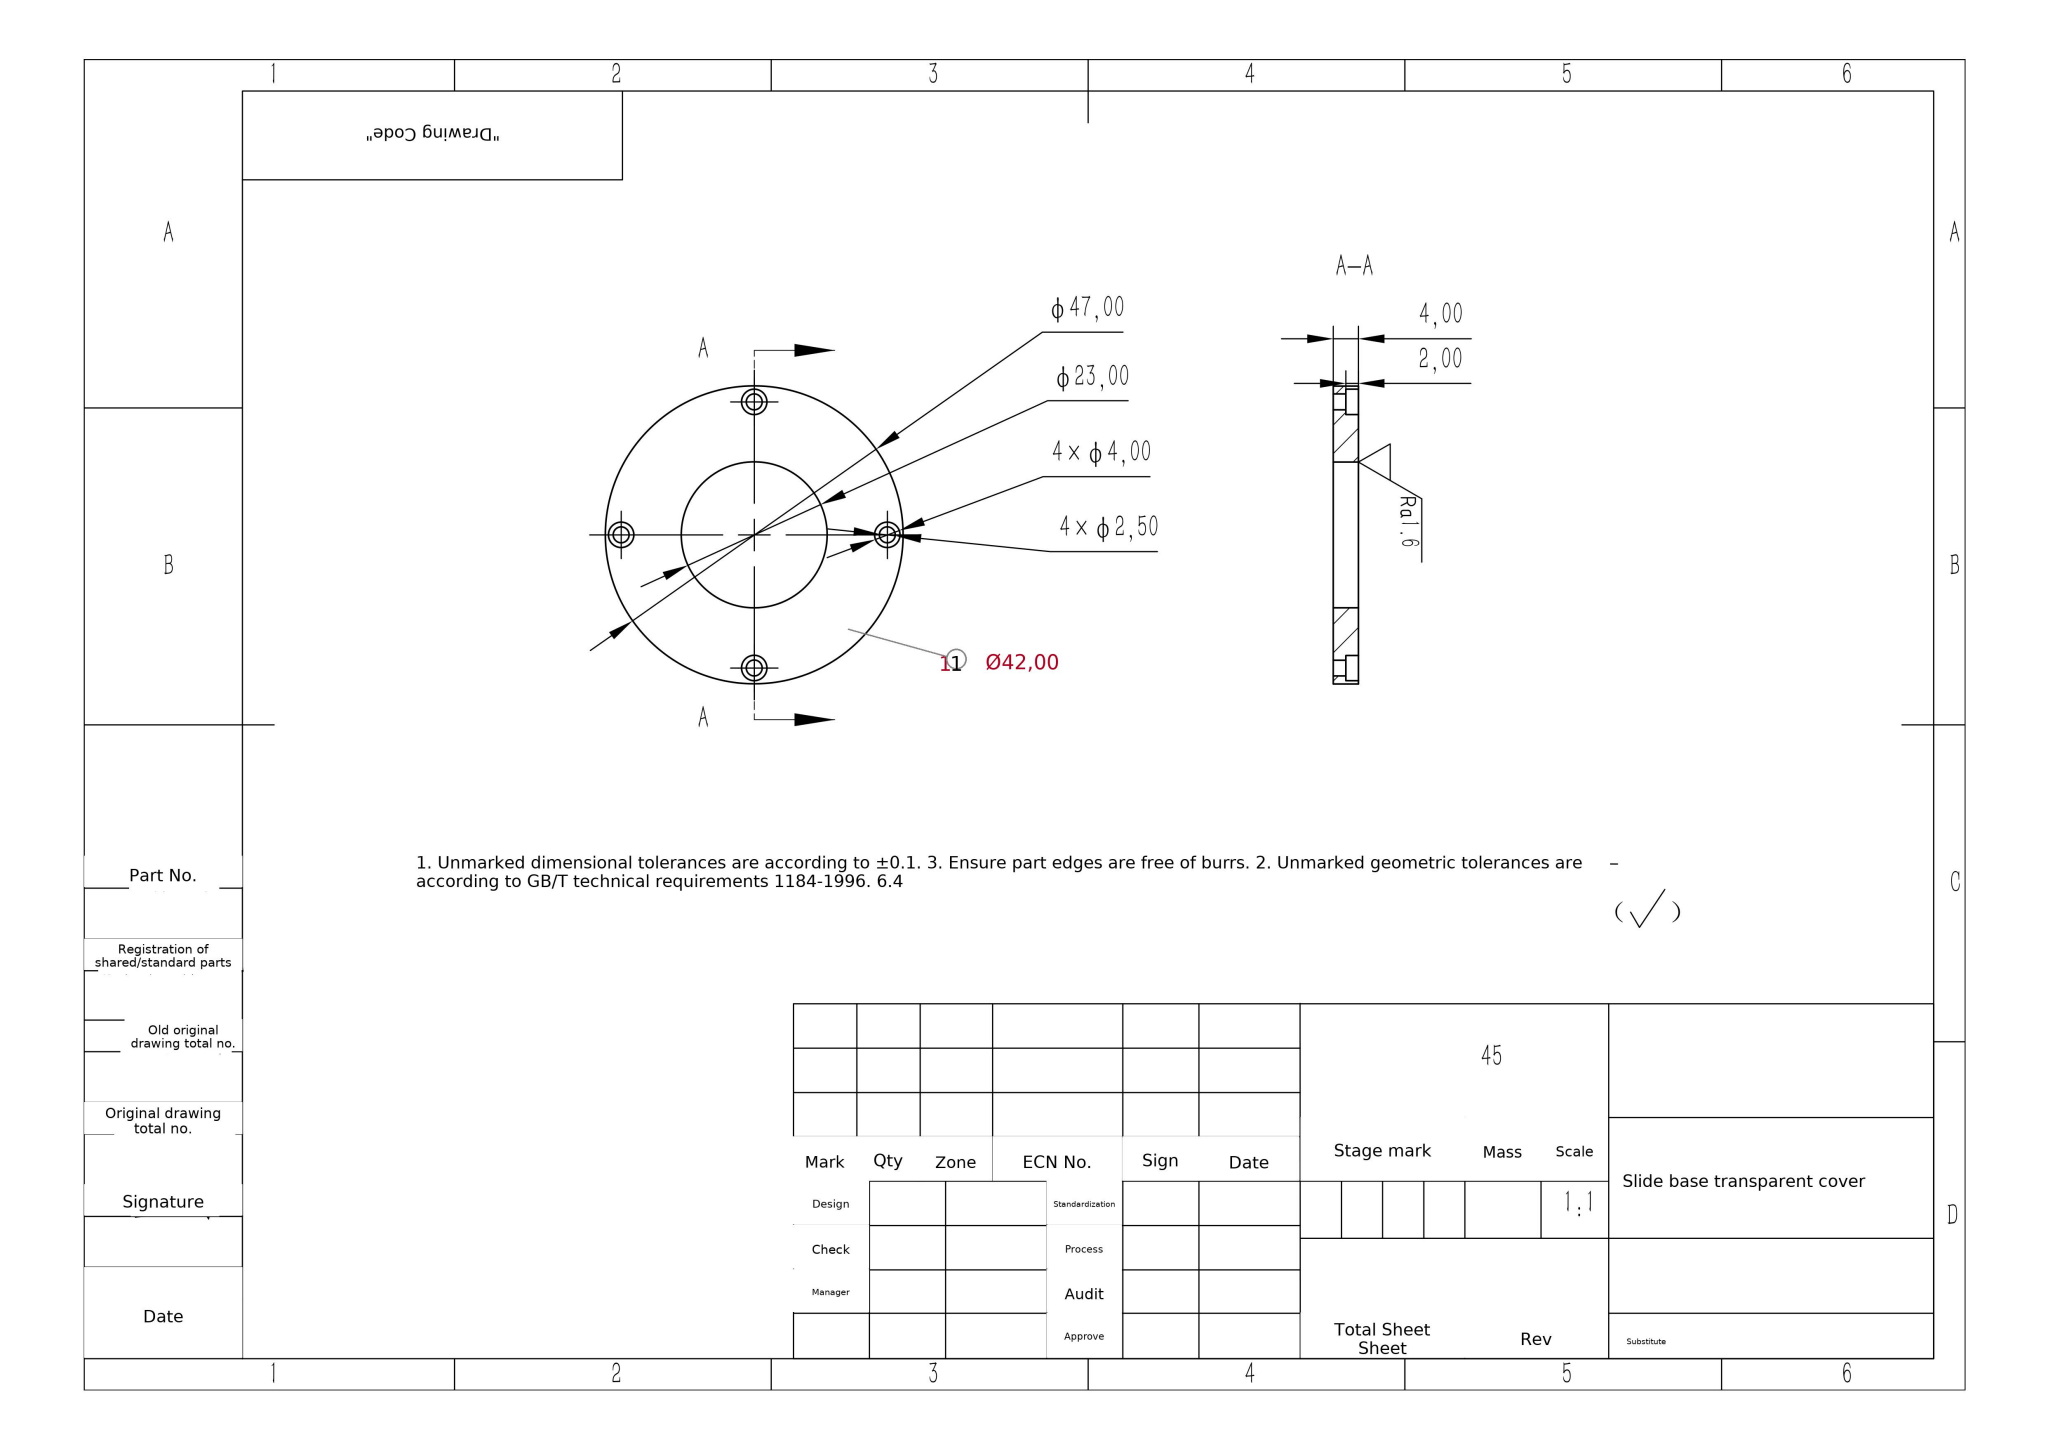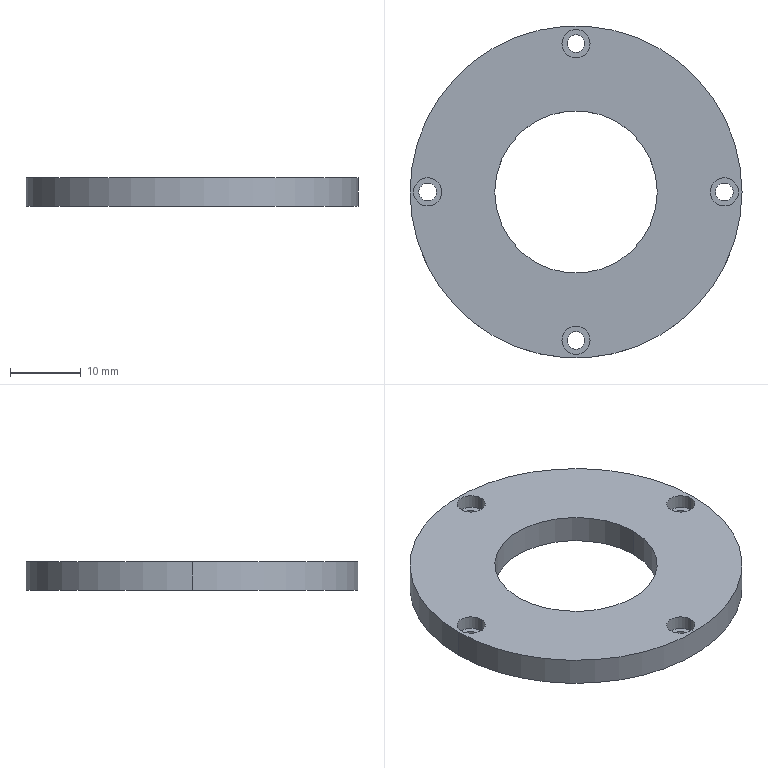Part | SolidWorks | mm | 1 solid | 26 faces | box 47 x 47 x 4 mm | volume 5138 mm3 | cylinder 20 | plane 6 | commonest cylinder face diameters 4 x8 2.5 x8 23 x2 47 x2
build123d program:
from build123d import *

# Parameters (mm, degrees)
SKETCH1_R           = 23.5
SKETCH1_R_2         = 11.5
SKETCH1_R_3         = 1.25
BOSS_EXTRUDE1_DEPTH = 4
SKETCH2_R           = 2
CUT_EXTRUDE1_DEPTH  = 2


with BuildPart() as part:
    # Sketch1 → Boss-Extrude1 (new body)
    with BuildSketch(Plane.XY):
        Circle(SKETCH1_R)
        Circle(SKETCH1_R_2, mode=Mode.SUBTRACT)
        with Locations((21, 0)):
            Circle(SKETCH1_R_3, mode=Mode.SUBTRACT)
        with Locations((0, -21)):
            Circle(SKETCH1_R_3, mode=Mode.SUBTRACT)
        with Locations((-21, 0)):
            Circle(SKETCH1_R_3, mode=Mode.SUBTRACT)
        with Locations((0, 21)):
            Circle(SKETCH1_R_3, mode=Mode.SUBTRACT)
    extrude(amount=BOSS_EXTRUDE1_DEPTH)

    # Sketch2 → Cut-Extrude1 (cut)
    with BuildSketch(Plane.XY.offset(4)):
        with Locations((0, 21)):
            Circle(SKETCH2_R)
        with Locations((21, 0)):
            Circle(SKETCH2_R)
        with Locations((0, -21)):
            Circle(SKETCH2_R)
        with Locations((-21, 0)):
            Circle(SKETCH2_R)
    extrude(amount=-CUT_EXTRUDE1_DEPTH, mode=Mode.SUBTRACT)


solid = part.part
STEP:
#1=CARTESIAN_POINT('',(19.,0.,2.));
#2=VERTEX_POINT('',#1);
#3=CARTESIAN_POINT('',(23.,0.,2.));
#4=VERTEX_POINT('',#3);
#5=CARTESIAN_POINT('',(21.,0.,2.));
#6=DIRECTION('',(0.,0.,1.));
#7=DIRECTION('',(1.,0.,0.));
#8=AXIS2_PLACEMENT_3D('',#5,#6,#7);
#9=CIRCLE('',#8,2.);
#10=EDGE_CURVE('',#2,#4,#9,.T.);
#11=ORIENTED_EDGE('',*,*,#10,.F.);
#12=CARTESIAN_POINT('',(19.,0.,4.));
#13=VERTEX_POINT('',#12);
#14=CARTESIAN_POINT('',(19.,0.,2.));
#15=DIRECTION('',(0.,0.,1.));
#16=VECTOR('',#15,1000.);
#17=LINE('',#14,#16);
#18=EDGE_CURVE('',#2,#13,#17,.T.);
#19=ORIENTED_EDGE('',*,*,#18,.T.);
#20=CARTESIAN_POINT('',(23.,0.,4.));
#21=VERTEX_POINT('',#20);
#22=CARTESIAN_POINT('',(21.,0.,4.));
#23=DIRECTION('',(0.,0.,1.));
#24=DIRECTION('',(1.,0.,0.));
#25=AXIS2_PLACEMENT_3D('',#22,#23,#24);
#26=CIRCLE('',#25,2.);
#27=EDGE_CURVE('',#13,#21,#26,.T.);
#28=ORIENTED_EDGE('',*,*,#27,.T.);
#29=CARTESIAN_POINT('',(23.,0.,2.));
#30=DIRECTION('',(0.,0.,1.));
#31=VECTOR('',#30,1000.);
#32=LINE('',#29,#31);
#33=EDGE_CURVE('',#4,#21,#32,.T.);
#34=ORIENTED_EDGE('',*,*,#33,.F.);
#35=EDGE_LOOP('',(#11,#19,#28,#34));
#36=FACE_OUTER_BOUND('',#35,.T.);
#37=CARTESIAN_POINT('',(21.,0.,2.));
#38=DIRECTION('',(0.,0.,1.));
#39=DIRECTION('',(1.,0.,0.));
#40=AXIS2_PLACEMENT_3D('',#37,#38,#39);
#41=CYLINDRICAL_SURFACE('',#40,2.);
#42=ADVANCED_FACE('',(#36),#41,.F.);
#43=CARTESIAN_POINT('',(-2.,-21.,2.));
#44=VERTEX_POINT('',#43);
#45=CARTESIAN_POINT('',(2.,-21.,2.));
#46=VERTEX_POINT('',#45);
#47=CARTESIAN_POINT('',(0.,-21.,2.));
#48=DIRECTION('',(0.,0.,1.));
#49=DIRECTION('',(1.,0.,0.));
#50=AXIS2_PLACEMENT_3D('',#47,#48,#49);
#51=CIRCLE('',#50,2.);
#52=EDGE_CURVE('',#44,#46,#51,.T.);
#53=ORIENTED_EDGE('',*,*,#52,.F.);
#54=CARTESIAN_POINT('',(-2.,-21.,4.));
#55=VERTEX_POINT('',#54);
#56=CARTESIAN_POINT('',(-2.,-21.,2.));
#57=DIRECTION('',(0.,0.,1.));
#58=VECTOR('',#57,1000.);
#59=LINE('',#56,#58);
#60=EDGE_CURVE('',#44,#55,#59,.T.);
#61=ORIENTED_EDGE('',*,*,#60,.T.);
#62=CARTESIAN_POINT('',(2.,-21.,4.));
#63=VERTEX_POINT('',#62);
#64=CARTESIAN_POINT('',(0.,-21.,4.));
#65=DIRECTION('',(0.,0.,1.));
#66=DIRECTION('',(1.,0.,0.));
#67=AXIS2_PLACEMENT_3D('',#64,#65,#66);
#68=CIRCLE('',#67,2.);
#69=EDGE_CURVE('',#55,#63,#68,.T.);
#70=ORIENTED_EDGE('',*,*,#69,.T.);
#71=CARTESIAN_POINT('',(2.,-21.,2.));
#72=DIRECTION('',(0.,0.,1.));
#73=VECTOR('',#72,1000.);
#74=LINE('',#71,#73);
#75=EDGE_CURVE('',#46,#63,#74,.T.);
#76=ORIENTED_EDGE('',*,*,#75,.F.);
#77=EDGE_LOOP('',(#53,#61,#70,#76));
#78=FACE_OUTER_BOUND('',#77,.T.);
#79=CARTESIAN_POINT('',(0.,-21.,2.));
#80=DIRECTION('',(0.,0.,1.));
#81=DIRECTION('',(1.,0.,0.));
#82=AXIS2_PLACEMENT_3D('',#79,#80,#81);
#83=CYLINDRICAL_SURFACE('',#82,2.);
#84=ADVANCED_FACE('',(#78),#83,.F.);
#85=CARTESIAN_POINT('',(-23.,-0.,2.));
#86=VERTEX_POINT('',#85);
#87=CARTESIAN_POINT('',(-19.,-0.,2.));
#88=VERTEX_POINT('',#87);
#89=CARTESIAN_POINT('',(-21.,-0.,2.));
#90=DIRECTION('',(0.,0.,1.));
#91=DIRECTION('',(1.,0.,0.));
#92=AXIS2_PLACEMENT_3D('',#89,#90,#91);
#93=CIRCLE('',#92,2.);
#94=EDGE_CURVE('',#86,#88,#93,.T.);
#95=ORIENTED_EDGE('',*,*,#94,.F.);
#96=CARTESIAN_POINT('',(-23.,-0.,4.));
#97=VERTEX_POINT('',#96);
#98=CARTESIAN_POINT('',(-23.,-0.,2.));
#99=DIRECTION('',(0.,0.,1.));
#100=VECTOR('',#99,1000.);
#101=LINE('',#98,#100);
#102=EDGE_CURVE('',#86,#97,#101,.T.);
#103=ORIENTED_EDGE('',*,*,#102,.T.);
#104=CARTESIAN_POINT('',(-19.,-0.,4.));
#105=VERTEX_POINT('',#104);
#106=CARTESIAN_POINT('',(-21.,-0.,4.));
#107=DIRECTION('',(0.,0.,1.));
#108=DIRECTION('',(1.,0.,0.));
#109=AXIS2_PLACEMENT_3D('',#106,#107,#108);
#110=CIRCLE('',#109,2.);
#111=EDGE_CURVE('',#97,#105,#110,.T.);
#112=ORIENTED_EDGE('',*,*,#111,.T.);
#113=CARTESIAN_POINT('',(-19.,-0.,2.));
#114=DIRECTION('',(0.,0.,1.));
#115=VECTOR('',#114,1000.);
#116=LINE('',#113,#115);
#117=EDGE_CURVE('',#88,#105,#116,.T.);
#118=ORIENTED_EDGE('',*,*,#117,.F.);
#119=EDGE_LOOP('',(#95,#103,#112,#118));
#120=FACE_OUTER_BOUND('',#119,.T.);
#121=CARTESIAN_POINT('',(-21.,-0.,2.));
#122=DIRECTION('',(0.,0.,1.));
#123=DIRECTION('',(1.,0.,0.));
#124=AXIS2_PLACEMENT_3D('',#121,#122,#123);
#125=CYLINDRICAL_SURFACE('',#124,2.);
#126=ADVANCED_FACE('',(#120),#125,.F.);
#127=CARTESIAN_POINT('',(-2.,21.,2.));
#128=VERTEX_POINT('',#127);
#129=CARTESIAN_POINT('',(2.,21.,2.));
#130=VERTEX_POINT('',#129);
#131=CARTESIAN_POINT('',(0.,21.,2.));
#132=DIRECTION('',(0.,0.,1.));
#133=DIRECTION('',(1.,0.,0.));
#134=AXIS2_PLACEMENT_3D('',#131,#132,#133);
#135=CIRCLE('',#134,2.);
#136=EDGE_CURVE('',#128,#130,#135,.T.);
#137=ORIENTED_EDGE('',*,*,#136,.F.);
#138=CARTESIAN_POINT('',(-2.,21.,4.));
#139=VERTEX_POINT('',#138);
#140=CARTESIAN_POINT('',(-2.,21.,2.));
#141=DIRECTION('',(0.,0.,1.));
#142=VECTOR('',#141,1000.);
#143=LINE('',#140,#142);
#144=EDGE_CURVE('',#128,#139,#143,.T.);
#145=ORIENTED_EDGE('',*,*,#144,.T.);
#146=CARTESIAN_POINT('',(2.,21.,4.));
#147=VERTEX_POINT('',#146);
#148=CARTESIAN_POINT('',(0.,21.,4.));
#149=DIRECTION('',(0.,0.,1.));
#150=DIRECTION('',(1.,0.,0.));
#151=AXIS2_PLACEMENT_3D('',#148,#149,#150);
#152=CIRCLE('',#151,2.);
#153=EDGE_CURVE('',#139,#147,#152,.T.);
#154=ORIENTED_EDGE('',*,*,#153,.T.);
#155=CARTESIAN_POINT('',(2.,21.,2.));
#156=DIRECTION('',(0.,0.,1.));
#157=VECTOR('',#156,1000.);
#158=LINE('',#155,#157);
#159=EDGE_CURVE('',#130,#147,#158,.T.);
#160=ORIENTED_EDGE('',*,*,#159,.F.);
#161=EDGE_LOOP('',(#137,#145,#154,#160));
#162=FACE_OUTER_BOUND('',#161,.T.);
#163=CARTESIAN_POINT('',(0.,21.,2.));
#164=DIRECTION('',(0.,0.,1.));
#165=DIRECTION('',(1.,0.,0.));
#166=AXIS2_PLACEMENT_3D('',#163,#164,#165);
#167=CYLINDRICAL_SURFACE('',#166,2.);
#168=ADVANCED_FACE('',(#162),#167,.F.);
#169=CARTESIAN_POINT('',(-11.5,0.,4.));
#170=VERTEX_POINT('',#169);
#171=CARTESIAN_POINT('',(11.5,0.,4.));
#172=VERTEX_POINT('',#171);
#173=CARTESIAN_POINT('',(0.,0.,4.));
#174=DIRECTION('',(0.,0.,1.));
#175=DIRECTION('',(1.,0.,0.));
#176=AXIS2_PLACEMENT_3D('',#173,#174,#175);
#177=CIRCLE('',#176,11.5);
#178=EDGE_CURVE('',#170,#172,#177,.T.);
#179=ORIENTED_EDGE('',*,*,#178,.T.);
#180=CARTESIAN_POINT('',(11.5,0.,0.));
#181=VERTEX_POINT('',#180);
#182=CARTESIAN_POINT('',(11.5,0.,4.));
#183=DIRECTION('',(0.,0.,-1.));
#184=VECTOR('',#183,1000.);
#185=LINE('',#182,#184);
#186=EDGE_CURVE('',#172,#181,#185,.T.);
#187=ORIENTED_EDGE('',*,*,#186,.T.);
#188=CARTESIAN_POINT('',(-11.5,0.,0.));
#189=VERTEX_POINT('',#188);
#190=CARTESIAN_POINT('',(0.,0.,0.));
#191=DIRECTION('',(0.,0.,1.));
#192=DIRECTION('',(1.,0.,0.));
#193=AXIS2_PLACEMENT_3D('',#190,#191,#192);
#194=CIRCLE('',#193,11.5);
#195=EDGE_CURVE('',#189,#181,#194,.T.);
#196=ORIENTED_EDGE('',*,*,#195,.F.);
#197=CARTESIAN_POINT('',(-11.5,0.,4.));
#198=DIRECTION('',(0.,0.,-1.));
#199=VECTOR('',#198,1000.);
#200=LINE('',#197,#199);
#201=EDGE_CURVE('',#170,#189,#200,.T.);
#202=ORIENTED_EDGE('',*,*,#201,.F.);
#203=EDGE_LOOP('',(#179,#187,#196,#202));
#204=FACE_OUTER_BOUND('',#203,.T.);
#205=CARTESIAN_POINT('',(0.,0.,4.));
#206=DIRECTION('',(0.,0.,-1.));
#207=DIRECTION('',(-1.,0.,0.));
#208=AXIS2_PLACEMENT_3D('',#205,#206,#207);
#209=CYLINDRICAL_SURFACE('',#208,11.5);
#210=ADVANCED_FACE('',(#204),#209,.F.);
#211=CARTESIAN_POINT('',(23.5,0.,4.));
#212=VERTEX_POINT('',#211);
#213=CARTESIAN_POINT('',(-23.5,0.,4.));
#214=VERTEX_POINT('',#213);
#215=CARTESIAN_POINT('',(0.,0.,4.));
#216=DIRECTION('',(0.,0.,1.));
#217=DIRECTION('',(1.,0.,0.));
#218=AXIS2_PLACEMENT_3D('',#215,#216,#217);
#219=CIRCLE('',#218,23.5);
#220=EDGE_CURVE('',#212,#214,#219,.T.);
#221=ORIENTED_EDGE('',*,*,#220,.F.);
#222=CARTESIAN_POINT('',(23.5,0.,0.));
#223=VERTEX_POINT('',#222);
#224=CARTESIAN_POINT('',(23.5,0.,4.));
#225=DIRECTION('',(0.,0.,-1.));
#226=VECTOR('',#225,1000.);
#227=LINE('',#224,#226);
#228=EDGE_CURVE('',#212,#223,#227,.T.);
#229=ORIENTED_EDGE('',*,*,#228,.T.);
#230=CARTESIAN_POINT('',(-23.5,0.,0.));
#231=VERTEX_POINT('',#230);
#232=CARTESIAN_POINT('',(0.,0.,0.));
#233=DIRECTION('',(0.,0.,1.));
#234=DIRECTION('',(1.,0.,0.));
#235=AXIS2_PLACEMENT_3D('',#232,#233,#234);
#236=CIRCLE('',#235,23.5);
#237=EDGE_CURVE('',#223,#231,#236,.T.);
#238=ORIENTED_EDGE('',*,*,#237,.T.);
#239=CARTESIAN_POINT('',(-23.5,0.,4.));
#240=DIRECTION('',(0.,0.,-1.));
#241=VECTOR('',#240,1000.);
#242=LINE('',#239,#241);
#243=EDGE_CURVE('',#214,#231,#242,.T.);
#244=ORIENTED_EDGE('',*,*,#243,.F.);
#245=EDGE_LOOP('',(#221,#229,#238,#244));
#246=FACE_OUTER_BOUND('',#245,.T.);
#247=CARTESIAN_POINT('',(0.,0.,4.));
#248=DIRECTION('',(0.,0.,-1.));
#249=DIRECTION('',(-1.,0.,0.));
#250=AXIS2_PLACEMENT_3D('',#247,#248,#249);
#251=CYLINDRICAL_SURFACE('',#250,23.5);
#252=ADVANCED_FACE('',(#246),#251,.T.);
#253=CARTESIAN_POINT('',(-1.25,21.,2.));
#254=VERTEX_POINT('',#253);
#255=CARTESIAN_POINT('',(1.25,21.,2.));
#256=VERTEX_POINT('',#255);
#257=CARTESIAN_POINT('',(0.,21.,2.));
#258=DIRECTION('',(0.,0.,1.));
#259=DIRECTION('',(1.,0.,0.));
#260=AXIS2_PLACEMENT_3D('',#257,#258,#259);
#261=CIRCLE('',#260,1.25);
#262=EDGE_CURVE('',#254,#256,#261,.T.);
#263=ORIENTED_EDGE('',*,*,#262,.T.);
#264=CARTESIAN_POINT('',(1.25,21.,0.));
#265=VERTEX_POINT('',#264);
#266=CARTESIAN_POINT('',(1.25,21.,4.));
#267=DIRECTION('',(0.,0.,-1.));
#268=VECTOR('',#267,1000.);
#269=LINE('',#266,#268);
#270=EDGE_CURVE('',#256,#265,#269,.T.);
#271=ORIENTED_EDGE('',*,*,#270,.T.);
#272=CARTESIAN_POINT('',(-1.25,21.,0.));
#273=VERTEX_POINT('',#272);
#274=CARTESIAN_POINT('',(0.,21.,0.));
#275=DIRECTION('',(0.,0.,1.));
#276=DIRECTION('',(1.,0.,0.));
#277=AXIS2_PLACEMENT_3D('',#274,#275,#276);
#278=CIRCLE('',#277,1.25);
#279=EDGE_CURVE('',#273,#265,#278,.T.);
#280=ORIENTED_EDGE('',*,*,#279,.F.);
#281=CARTESIAN_POINT('',(-1.25,21.,4.));
#282=DIRECTION('',(0.,0.,-1.));
#283=VECTOR('',#282,1000.);
#284=LINE('',#281,#283);
#285=EDGE_CURVE('',#254,#273,#284,.T.);
#286=ORIENTED_EDGE('',*,*,#285,.F.);
#287=EDGE_LOOP('',(#263,#271,#280,#286));
#288=FACE_OUTER_BOUND('',#287,.T.);
#289=CARTESIAN_POINT('',(0.,21.,4.));
#290=DIRECTION('',(0.,0.,-1.));
#291=DIRECTION('',(-1.,0.,0.));
#292=AXIS2_PLACEMENT_3D('',#289,#290,#291);
#293=CYLINDRICAL_SURFACE('',#292,1.25);
#294=ADVANCED_FACE('',(#288),#293,.F.);
#295=CARTESIAN_POINT('',(-22.25,0.,2.));
#296=VERTEX_POINT('',#295);
#297=CARTESIAN_POINT('',(-19.75,0.,2.));
#298=VERTEX_POINT('',#297);
#299=CARTESIAN_POINT('',(-21.,0.,2.));
#300=DIRECTION('',(0.,0.,1.));
#301=DIRECTION('',(1.,0.,0.));
#302=AXIS2_PLACEMENT_3D('',#299,#300,#301);
#303=CIRCLE('',#302,1.25);
#304=EDGE_CURVE('',#296,#298,#303,.T.);
#305=ORIENTED_EDGE('',*,*,#304,.T.);
#306=CARTESIAN_POINT('',(-19.75,0.,0.));
#307=VERTEX_POINT('',#306);
#308=CARTESIAN_POINT('',(-19.75,0.,4.));
#309=DIRECTION('',(0.,0.,-1.));
#310=VECTOR('',#309,1000.);
#311=LINE('',#308,#310);
#312=EDGE_CURVE('',#298,#307,#311,.T.);
#313=ORIENTED_EDGE('',*,*,#312,.T.);
#314=CARTESIAN_POINT('',(-22.25,0.,0.));
#315=VERTEX_POINT('',#314);
#316=CARTESIAN_POINT('',(-21.,0.,0.));
#317=DIRECTION('',(0.,0.,1.));
#318=DIRECTION('',(1.,0.,0.));
#319=AXIS2_PLACEMENT_3D('',#316,#317,#318);
#320=CIRCLE('',#319,1.25);
#321=EDGE_CURVE('',#315,#307,#320,.T.);
#322=ORIENTED_EDGE('',*,*,#321,.F.);
#323=CARTESIAN_POINT('',(-22.25,0.,4.));
#324=DIRECTION('',(0.,0.,-1.));
#325=VECTOR('',#324,1000.);
#326=LINE('',#323,#325);
#327=EDGE_CURVE('',#296,#315,#326,.T.);
#328=ORIENTED_EDGE('',*,*,#327,.F.);
#329=EDGE_LOOP('',(#305,#313,#322,#328));
#330=FACE_OUTER_BOUND('',#329,.T.);
#331=CARTESIAN_POINT('',(-21.,0.,4.));
#332=DIRECTION('',(0.,0.,-1.));
#333=DIRECTION('',(-1.,0.,0.));
#334=AXIS2_PLACEMENT_3D('',#331,#332,#333);
#335=CYLINDRICAL_SURFACE('',#334,1.25);
#336=ADVANCED_FACE('',(#330),#335,.F.);
#337=CARTESIAN_POINT('',(-1.25,-21.,2.));
#338=VERTEX_POINT('',#337);
#339=CARTESIAN_POINT('',(1.25,-21.,2.));
#340=VERTEX_POINT('',#339);
#341=CARTESIAN_POINT('',(-0.,-21.,2.));
#342=DIRECTION('',(0.,0.,1.));
#343=DIRECTION('',(1.,0.,0.));
#344=AXIS2_PLACEMENT_3D('',#341,#342,#343);
#345=CIRCLE('',#344,1.25);
#346=EDGE_CURVE('',#338,#340,#345,.T.);
#347=ORIENTED_EDGE('',*,*,#346,.T.);
#348=CARTESIAN_POINT('',(1.25,-21.,0.));
#349=VERTEX_POINT('',#348);
#350=CARTESIAN_POINT('',(1.25,-21.,4.));
#351=DIRECTION('',(0.,0.,-1.));
#352=VECTOR('',#351,1000.);
#353=LINE('',#350,#352);
#354=EDGE_CURVE('',#340,#349,#353,.T.);
#355=ORIENTED_EDGE('',*,*,#354,.T.);
#356=CARTESIAN_POINT('',(-1.25,-21.,0.));
#357=VERTEX_POINT('',#356);
#358=CARTESIAN_POINT('',(-0.,-21.,0.));
#359=DIRECTION('',(0.,0.,1.));
#360=DIRECTION('',(1.,0.,0.));
#361=AXIS2_PLACEMENT_3D('',#358,#359,#360);
#362=CIRCLE('',#361,1.25);
#363=EDGE_CURVE('',#357,#349,#362,.T.);
#364=ORIENTED_EDGE('',*,*,#363,.F.);
#365=CARTESIAN_POINT('',(-1.25,-21.,4.));
#366=DIRECTION('',(0.,0.,-1.));
#367=VECTOR('',#366,1000.);
#368=LINE('',#365,#367);
#369=EDGE_CURVE('',#338,#357,#368,.T.);
#370=ORIENTED_EDGE('',*,*,#369,.F.);
#371=EDGE_LOOP('',(#347,#355,#364,#370));
#372=FACE_OUTER_BOUND('',#371,.T.);
#373=CARTESIAN_POINT('',(-0.,-21.,4.));
#374=DIRECTION('',(0.,0.,-1.));
#375=DIRECTION('',(-1.,0.,0.));
#376=AXIS2_PLACEMENT_3D('',#373,#374,#375);
#377=CYLINDRICAL_SURFACE('',#376,1.25);
#378=ADVANCED_FACE('',(#372),#377,.F.);
#379=CARTESIAN_POINT('',(19.75,0.,2.));
#380=VERTEX_POINT('',#379);
#381=CARTESIAN_POINT('',(22.25,0.,2.));
#382=VERTEX_POINT('',#381);
#383=CARTESIAN_POINT('',(21.,0.,2.));
#384=DIRECTION('',(0.,0.,1.));
#385=DIRECTION('',(1.,0.,0.));
#386=AXIS2_PLACEMENT_3D('',#383,#384,#385);
#387=CIRCLE('',#386,1.25);
#388=EDGE_CURVE('',#380,#382,#387,.T.);
#389=ORIENTED_EDGE('',*,*,#388,.T.);
#390=CARTESIAN_POINT('',(22.25,0.,0.));
#391=VERTEX_POINT('',#390);
#392=CARTESIAN_POINT('',(22.25,0.,4.));
#393=DIRECTION('',(0.,0.,-1.));
#394=VECTOR('',#393,1000.);
#395=LINE('',#392,#394);
#396=EDGE_CURVE('',#382,#391,#395,.T.);
#397=ORIENTED_EDGE('',*,*,#396,.T.);
#398=CARTESIAN_POINT('',(19.75,0.,0.));
#399=VERTEX_POINT('',#398);
#400=CARTESIAN_POINT('',(21.,0.,0.));
#401=DIRECTION('',(0.,0.,1.));
#402=DIRECTION('',(1.,0.,0.));
#403=AXIS2_PLACEMENT_3D('',#400,#401,#402);
#404=CIRCLE('',#403,1.25);
#405=EDGE_CURVE('',#399,#391,#404,.T.);
#406=ORIENTED_EDGE('',*,*,#405,.F.);
#407=CARTESIAN_POINT('',(19.75,0.,4.));
#408=DIRECTION('',(0.,0.,-1.));
#409=VECTOR('',#408,1000.);
#410=LINE('',#407,#409);
#411=EDGE_CURVE('',#380,#399,#410,.T.);
#412=ORIENTED_EDGE('',*,*,#411,.F.);
#413=EDGE_LOOP('',(#389,#397,#406,#412));
#414=FACE_OUTER_BOUND('',#413,.T.);
#415=CARTESIAN_POINT('',(21.,0.,4.));
#416=DIRECTION('',(0.,0.,-1.));
#417=DIRECTION('',(-1.,0.,0.));
#418=AXIS2_PLACEMENT_3D('',#415,#416,#417);
#419=CYLINDRICAL_SURFACE('',#418,1.25);
#420=ADVANCED_FACE('',(#414),#419,.F.);
#421=ORIENTED_EDGE('',*,*,#396,.F.);
#422=CARTESIAN_POINT('',(21.,0.,2.));
#423=DIRECTION('',(0.,0.,1.));
#424=DIRECTION('',(1.,0.,0.));
#425=AXIS2_PLACEMENT_3D('',#422,#423,#424);
#426=CIRCLE('',#425,1.25);
#427=EDGE_CURVE('',#382,#380,#426,.T.);
#428=ORIENTED_EDGE('',*,*,#427,.T.);
#429=ORIENTED_EDGE('',*,*,#411,.T.);
#430=CARTESIAN_POINT('',(21.,0.,0.));
#431=DIRECTION('',(0.,0.,1.));
#432=DIRECTION('',(1.,0.,0.));
#433=AXIS2_PLACEMENT_3D('',#430,#431,#432);
#434=CIRCLE('',#433,1.25);
#435=EDGE_CURVE('',#391,#399,#434,.T.);
#436=ORIENTED_EDGE('',*,*,#435,.F.);
#437=EDGE_LOOP('',(#421,#428,#429,#436));
#438=FACE_OUTER_BOUND('',#437,.T.);
#439=CARTESIAN_POINT('',(21.,0.,4.));
#440=DIRECTION('',(0.,0.,-1.));
#441=DIRECTION('',(-1.,0.,0.));
#442=AXIS2_PLACEMENT_3D('',#439,#440,#441);
#443=CYLINDRICAL_SURFACE('',#442,1.25);
#444=ADVANCED_FACE('',(#438),#443,.F.);
#445=ORIENTED_EDGE('',*,*,#354,.F.);
#446=CARTESIAN_POINT('',(-0.,-21.,2.));
#447=DIRECTION('',(0.,0.,1.));
#448=DIRECTION('',(1.,0.,0.));
#449=AXIS2_PLACEMENT_3D('',#446,#447,#448);
#450=CIRCLE('',#449,1.25);
#451=EDGE_CURVE('',#340,#338,#450,.T.);
#452=ORIENTED_EDGE('',*,*,#451,.T.);
#453=ORIENTED_EDGE('',*,*,#369,.T.);
#454=CARTESIAN_POINT('',(-0.,-21.,0.));
#455=DIRECTION('',(0.,0.,1.));
#456=DIRECTION('',(1.,0.,0.));
#457=AXIS2_PLACEMENT_3D('',#454,#455,#456);
#458=CIRCLE('',#457,1.25);
#459=EDGE_CURVE('',#349,#357,#458,.T.);
#460=ORIENTED_EDGE('',*,*,#459,.F.);
#461=EDGE_LOOP('',(#445,#452,#453,#460));
#462=FACE_OUTER_BOUND('',#461,.T.);
#463=CARTESIAN_POINT('',(-0.,-21.,4.));
#464=DIRECTION('',(0.,0.,-1.));
#465=DIRECTION('',(-1.,0.,0.));
#466=AXIS2_PLACEMENT_3D('',#463,#464,#465);
#467=CYLINDRICAL_SURFACE('',#466,1.25);
#468=ADVANCED_FACE('',(#462),#467,.F.);
#469=ORIENTED_EDGE('',*,*,#312,.F.);
#470=CARTESIAN_POINT('',(-21.,0.,2.));
#471=DIRECTION('',(0.,0.,1.));
#472=DIRECTION('',(1.,0.,0.));
#473=AXIS2_PLACEMENT_3D('',#470,#471,#472);
#474=CIRCLE('',#473,1.25);
#475=EDGE_CURVE('',#298,#296,#474,.T.);
#476=ORIENTED_EDGE('',*,*,#475,.T.);
#477=ORIENTED_EDGE('',*,*,#327,.T.);
#478=CARTESIAN_POINT('',(-21.,0.,0.));
#479=DIRECTION('',(0.,0.,1.));
#480=DIRECTION('',(1.,0.,0.));
#481=AXIS2_PLACEMENT_3D('',#478,#479,#480);
#482=CIRCLE('',#481,1.25);
#483=EDGE_CURVE('',#307,#315,#482,.T.);
#484=ORIENTED_EDGE('',*,*,#483,.F.);
#485=EDGE_LOOP('',(#469,#476,#477,#484));
#486=FACE_OUTER_BOUND('',#485,.T.);
#487=CARTESIAN_POINT('',(-21.,0.,4.));
#488=DIRECTION('',(0.,0.,-1.));
#489=DIRECTION('',(-1.,0.,0.));
#490=AXIS2_PLACEMENT_3D('',#487,#488,#489);
#491=CYLINDRICAL_SURFACE('',#490,1.25);
#492=ADVANCED_FACE('',(#486),#491,.F.);
#493=ORIENTED_EDGE('',*,*,#270,.F.);
#494=CARTESIAN_POINT('',(0.,21.,2.));
#495=DIRECTION('',(0.,0.,1.));
#496=DIRECTION('',(1.,0.,0.));
#497=AXIS2_PLACEMENT_3D('',#494,#495,#496);
#498=CIRCLE('',#497,1.25);
#499=EDGE_CURVE('',#256,#254,#498,.T.);
#500=ORIENTED_EDGE('',*,*,#499,.T.);
#501=ORIENTED_EDGE('',*,*,#285,.T.);
#502=CARTESIAN_POINT('',(0.,21.,0.));
#503=DIRECTION('',(0.,0.,1.));
#504=DIRECTION('',(1.,0.,0.));
#505=AXIS2_PLACEMENT_3D('',#502,#503,#504);
#506=CIRCLE('',#505,1.25);
#507=EDGE_CURVE('',#265,#273,#506,.T.);
#508=ORIENTED_EDGE('',*,*,#507,.F.);
#509=EDGE_LOOP('',(#493,#500,#501,#508));
#510=FACE_OUTER_BOUND('',#509,.T.);
#511=CARTESIAN_POINT('',(0.,21.,4.));
#512=DIRECTION('',(0.,0.,-1.));
#513=DIRECTION('',(-1.,0.,0.));
#514=AXIS2_PLACEMENT_3D('',#511,#512,#513);
#515=CYLINDRICAL_SURFACE('',#514,1.25);
#516=ADVANCED_FACE('',(#510),#515,.F.);
#517=CARTESIAN_POINT('',(21.,0.,4.));
#518=DIRECTION('',(0.,0.,1.));
#519=DIRECTION('',(1.,0.,0.));
#520=AXIS2_PLACEMENT_3D('',#517,#518,#519);
#521=CIRCLE('',#520,2.);
#522=EDGE_CURVE('',#21,#13,#521,.T.);
#523=ORIENTED_EDGE('',*,*,#522,.F.);
#524=ORIENTED_EDGE('',*,*,#27,.F.);
#525=EDGE_LOOP('',(#523,#524));
#526=FACE_BOUND('',#525,.T.);
#527=CARTESIAN_POINT('',(0.,-21.,4.));
#528=DIRECTION('',(0.,0.,1.));
#529=DIRECTION('',(1.,0.,0.));
#530=AXIS2_PLACEMENT_3D('',#527,#528,#529);
#531=CIRCLE('',#530,2.);
#532=EDGE_CURVE('',#63,#55,#531,.T.);
#533=ORIENTED_EDGE('',*,*,#532,.F.);
#534=ORIENTED_EDGE('',*,*,#69,.F.);
#535=EDGE_LOOP('',(#533,#534));
#536=FACE_BOUND('',#535,.T.);
#537=CARTESIAN_POINT('',(-21.,-0.,4.));
#538=DIRECTION('',(0.,0.,1.));
#539=DIRECTION('',(1.,0.,0.));
#540=AXIS2_PLACEMENT_3D('',#537,#538,#539);
#541=CIRCLE('',#540,2.);
#542=EDGE_CURVE('',#105,#97,#541,.T.);
#543=ORIENTED_EDGE('',*,*,#542,.F.);
#544=ORIENTED_EDGE('',*,*,#111,.F.);
#545=EDGE_LOOP('',(#543,#544));
#546=FACE_BOUND('',#545,.T.);
#547=CARTESIAN_POINT('',(0.,21.,4.));
#548=DIRECTION('',(0.,0.,1.));
#549=DIRECTION('',(1.,0.,0.));
#550=AXIS2_PLACEMENT_3D('',#547,#548,#549);
#551=CIRCLE('',#550,2.);
#552=EDGE_CURVE('',#147,#139,#551,.T.);
#553=ORIENTED_EDGE('',*,*,#552,.F.);
#554=ORIENTED_EDGE('',*,*,#153,.F.);
#555=EDGE_LOOP('',(#553,#554));
#556=FACE_BOUND('',#555,.T.);
#557=CARTESIAN_POINT('',(0.,0.,4.));
#558=DIRECTION('',(0.,0.,1.));
#559=DIRECTION('',(1.,0.,0.));
#560=AXIS2_PLACEMENT_3D('',#557,#558,#559);
#561=CIRCLE('',#560,23.5);
#562=EDGE_CURVE('',#214,#212,#561,.T.);
#563=ORIENTED_EDGE('',*,*,#562,.T.);
#564=ORIENTED_EDGE('',*,*,#220,.T.);
#565=EDGE_LOOP('',(#563,#564));
#566=FACE_OUTER_BOUND('',#565,.T.);
#567=ORIENTED_EDGE('',*,*,#178,.F.);
#568=CARTESIAN_POINT('',(0.,0.,4.));
#569=DIRECTION('',(0.,0.,1.));
#570=DIRECTION('',(1.,0.,0.));
#571=AXIS2_PLACEMENT_3D('',#568,#569,#570);
#572=CIRCLE('',#571,11.5);
#573=EDGE_CURVE('',#172,#170,#572,.T.);
#574=ORIENTED_EDGE('',*,*,#573,.F.);
#575=EDGE_LOOP('',(#567,#574));
#576=FACE_BOUND('',#575,.T.);
#577=CARTESIAN_POINT('',(0.,0.,4.));
#578=DIRECTION('',(0.,0.,1.));
#579=DIRECTION('',(1.,0.,0.));
#580=AXIS2_PLACEMENT_3D('',#577,#578,#579);
#581=PLANE('',#580);
#582=ADVANCED_FACE('',(#526,#536,#546,#556,#566,#576),#581,.T.);
#583=CARTESIAN_POINT('',(0.,0.,0.));
#584=DIRECTION('',(0.,0.,1.));
#585=DIRECTION('',(1.,0.,0.));
#586=AXIS2_PLACEMENT_3D('',#583,#584,#585);
#587=CIRCLE('',#586,23.5);
#588=EDGE_CURVE('',#231,#223,#587,.T.);
#589=ORIENTED_EDGE('',*,*,#588,.F.);
#590=ORIENTED_EDGE('',*,*,#237,.F.);
#591=EDGE_LOOP('',(#589,#590));
#592=FACE_OUTER_BOUND('',#591,.T.);
#593=ORIENTED_EDGE('',*,*,#195,.T.);
#594=CARTESIAN_POINT('',(0.,0.,0.));
#595=DIRECTION('',(0.,0.,1.));
#596=DIRECTION('',(1.,0.,0.));
#597=AXIS2_PLACEMENT_3D('',#594,#595,#596);
#598=CIRCLE('',#597,11.5);
#599=EDGE_CURVE('',#181,#189,#598,.T.);
#600=ORIENTED_EDGE('',*,*,#599,.T.);
#601=EDGE_LOOP('',(#593,#600));
#602=FACE_BOUND('',#601,.T.);
#603=ORIENTED_EDGE('',*,*,#405,.T.);
#604=ORIENTED_EDGE('',*,*,#435,.T.);
#605=EDGE_LOOP('',(#603,#604));
#606=FACE_BOUND('',#605,.T.);
#607=ORIENTED_EDGE('',*,*,#363,.T.);
#608=ORIENTED_EDGE('',*,*,#459,.T.);
#609=EDGE_LOOP('',(#607,#608));
#610=FACE_BOUND('',#609,.T.);
#611=ORIENTED_EDGE('',*,*,#321,.T.);
#612=ORIENTED_EDGE('',*,*,#483,.T.);
#613=EDGE_LOOP('',(#611,#612));
#614=FACE_BOUND('',#613,.T.);
#615=ORIENTED_EDGE('',*,*,#279,.T.);
#616=ORIENTED_EDGE('',*,*,#507,.T.);
#617=EDGE_LOOP('',(#615,#616));
#618=FACE_BOUND('',#617,.T.);
#619=CARTESIAN_POINT('',(0.,0.,0.));
#620=DIRECTION('',(0.,0.,1.));
#621=DIRECTION('',(1.,0.,0.));
#622=AXIS2_PLACEMENT_3D('',#619,#620,#621);
#623=PLANE('',#622);
#624=ADVANCED_FACE('',(#592,#602,#606,#610,#614,#618),#623,.F.);
#625=ORIENTED_EDGE('',*,*,#228,.F.);
#626=ORIENTED_EDGE('',*,*,#562,.F.);
#627=ORIENTED_EDGE('',*,*,#243,.T.);
#628=ORIENTED_EDGE('',*,*,#588,.T.);
#629=EDGE_LOOP('',(#625,#626,#627,#628));
#630=FACE_OUTER_BOUND('',#629,.T.);
#631=CARTESIAN_POINT('',(0.,0.,4.));
#632=DIRECTION('',(0.,0.,-1.));
#633=DIRECTION('',(-1.,0.,0.));
#634=AXIS2_PLACEMENT_3D('',#631,#632,#633);
#635=CYLINDRICAL_SURFACE('',#634,23.5);
#636=ADVANCED_FACE('',(#630),#635,.T.);
#637=ORIENTED_EDGE('',*,*,#186,.F.);
#638=ORIENTED_EDGE('',*,*,#573,.T.);
#639=ORIENTED_EDGE('',*,*,#201,.T.);
#640=ORIENTED_EDGE('',*,*,#599,.F.);
#641=EDGE_LOOP('',(#637,#638,#639,#640));
#642=FACE_OUTER_BOUND('',#641,.T.);
#643=CARTESIAN_POINT('',(0.,0.,4.));
#644=DIRECTION('',(0.,0.,-1.));
#645=DIRECTION('',(-1.,0.,0.));
#646=AXIS2_PLACEMENT_3D('',#643,#644,#645);
#647=CYLINDRICAL_SURFACE('',#646,11.5);
#648=ADVANCED_FACE('',(#642),#647,.F.);
#649=ORIENTED_EDGE('',*,*,#144,.F.);
#650=CARTESIAN_POINT('',(0.,21.,2.));
#651=DIRECTION('',(0.,0.,1.));
#652=DIRECTION('',(1.,0.,0.));
#653=AXIS2_PLACEMENT_3D('',#650,#651,#652);
#654=CIRCLE('',#653,2.);
#655=EDGE_CURVE('',#130,#128,#654,.T.);
#656=ORIENTED_EDGE('',*,*,#655,.F.);
#657=ORIENTED_EDGE('',*,*,#159,.T.);
#658=ORIENTED_EDGE('',*,*,#552,.T.);
#659=EDGE_LOOP('',(#649,#656,#657,#658));
#660=FACE_OUTER_BOUND('',#659,.T.);
#661=CARTESIAN_POINT('',(0.,21.,2.));
#662=DIRECTION('',(0.,0.,1.));
#663=DIRECTION('',(1.,0.,0.));
#664=AXIS2_PLACEMENT_3D('',#661,#662,#663);
#665=CYLINDRICAL_SURFACE('',#664,2.);
#666=ADVANCED_FACE('',(#660),#665,.F.);
#667=ORIENTED_EDGE('',*,*,#262,.F.);
#668=ORIENTED_EDGE('',*,*,#499,.F.);
#669=EDGE_LOOP('',(#667,#668));
#670=FACE_BOUND('',#669,.T.);
#671=ORIENTED_EDGE('',*,*,#655,.T.);
#672=ORIENTED_EDGE('',*,*,#136,.T.);
#673=EDGE_LOOP('',(#671,#672));
#674=FACE_OUTER_BOUND('',#673,.T.);
#675=CARTESIAN_POINT('',(0.,21.,2.));
#676=DIRECTION('',(0.,0.,1.));
#677=DIRECTION('',(1.,0.,0.));
#678=AXIS2_PLACEMENT_3D('',#675,#676,#677);
#679=PLANE('',#678);
#680=ADVANCED_FACE('',(#670,#674),#679,.T.);
#681=ORIENTED_EDGE('',*,*,#102,.F.);
#682=CARTESIAN_POINT('',(-21.,-0.,2.));
#683=DIRECTION('',(0.,0.,1.));
#684=DIRECTION('',(1.,0.,0.));
#685=AXIS2_PLACEMENT_3D('',#682,#683,#684);
#686=CIRCLE('',#685,2.);
#687=EDGE_CURVE('',#88,#86,#686,.T.);
#688=ORIENTED_EDGE('',*,*,#687,.F.);
#689=ORIENTED_EDGE('',*,*,#117,.T.);
#690=ORIENTED_EDGE('',*,*,#542,.T.);
#691=EDGE_LOOP('',(#681,#688,#689,#690));
#692=FACE_OUTER_BOUND('',#691,.T.);
#693=CARTESIAN_POINT('',(-21.,-0.,2.));
#694=DIRECTION('',(0.,0.,1.));
#695=DIRECTION('',(1.,0.,0.));
#696=AXIS2_PLACEMENT_3D('',#693,#694,#695);
#697=CYLINDRICAL_SURFACE('',#696,2.);
#698=ADVANCED_FACE('',(#692),#697,.F.);
#699=ORIENTED_EDGE('',*,*,#304,.F.);
#700=ORIENTED_EDGE('',*,*,#475,.F.);
#701=EDGE_LOOP('',(#699,#700));
#702=FACE_BOUND('',#701,.T.);
#703=ORIENTED_EDGE('',*,*,#687,.T.);
#704=ORIENTED_EDGE('',*,*,#94,.T.);
#705=EDGE_LOOP('',(#703,#704));
#706=FACE_OUTER_BOUND('',#705,.T.);
#707=CARTESIAN_POINT('',(-21.,-0.,2.));
#708=DIRECTION('',(0.,0.,1.));
#709=DIRECTION('',(1.,0.,0.));
#710=AXIS2_PLACEMENT_3D('',#707,#708,#709);
#711=PLANE('',#710);
#712=ADVANCED_FACE('',(#702,#706),#711,.T.);
#713=ORIENTED_EDGE('',*,*,#60,.F.);
#714=CARTESIAN_POINT('',(0.,-21.,2.));
#715=DIRECTION('',(0.,0.,1.));
#716=DIRECTION('',(1.,0.,0.));
#717=AXIS2_PLACEMENT_3D('',#714,#715,#716);
#718=CIRCLE('',#717,2.);
#719=EDGE_CURVE('',#46,#44,#718,.T.);
#720=ORIENTED_EDGE('',*,*,#719,.F.);
#721=ORIENTED_EDGE('',*,*,#75,.T.);
#722=ORIENTED_EDGE('',*,*,#532,.T.);
#723=EDGE_LOOP('',(#713,#720,#721,#722));
#724=FACE_OUTER_BOUND('',#723,.T.);
#725=CARTESIAN_POINT('',(0.,-21.,2.));
#726=DIRECTION('',(0.,0.,1.));
#727=DIRECTION('',(1.,0.,0.));
#728=AXIS2_PLACEMENT_3D('',#725,#726,#727);
#729=CYLINDRICAL_SURFACE('',#728,2.);
#730=ADVANCED_FACE('',(#724),#729,.F.);
#731=ORIENTED_EDGE('',*,*,#346,.F.);
#732=ORIENTED_EDGE('',*,*,#451,.F.);
#733=EDGE_LOOP('',(#731,#732));
#734=FACE_BOUND('',#733,.T.);
#735=ORIENTED_EDGE('',*,*,#719,.T.);
#736=ORIENTED_EDGE('',*,*,#52,.T.);
#737=EDGE_LOOP('',(#735,#736));
#738=FACE_OUTER_BOUND('',#737,.T.);
#739=CARTESIAN_POINT('',(0.,-21.,2.));
#740=DIRECTION('',(0.,0.,1.));
#741=DIRECTION('',(1.,0.,0.));
#742=AXIS2_PLACEMENT_3D('',#739,#740,#741);
#743=PLANE('',#742);
#744=ADVANCED_FACE('',(#734,#738),#743,.T.);
#745=ORIENTED_EDGE('',*,*,#18,.F.);
#746=CARTESIAN_POINT('',(21.,0.,2.));
#747=DIRECTION('',(0.,0.,1.));
#748=DIRECTION('',(1.,0.,0.));
#749=AXIS2_PLACEMENT_3D('',#746,#747,#748);
#750=CIRCLE('',#749,2.);
#751=EDGE_CURVE('',#4,#2,#750,.T.);
#752=ORIENTED_EDGE('',*,*,#751,.F.);
#753=ORIENTED_EDGE('',*,*,#33,.T.);
#754=ORIENTED_EDGE('',*,*,#522,.T.);
#755=EDGE_LOOP('',(#745,#752,#753,#754));
#756=FACE_OUTER_BOUND('',#755,.T.);
#757=CARTESIAN_POINT('',(21.,0.,2.));
#758=DIRECTION('',(0.,0.,1.));
#759=DIRECTION('',(1.,0.,0.));
#760=AXIS2_PLACEMENT_3D('',#757,#758,#759);
#761=CYLINDRICAL_SURFACE('',#760,2.);
#762=ADVANCED_FACE('',(#756),#761,.F.);
#763=ORIENTED_EDGE('',*,*,#388,.F.);
#764=ORIENTED_EDGE('',*,*,#427,.F.);
#765=EDGE_LOOP('',(#763,#764));
#766=FACE_BOUND('',#765,.T.);
#767=ORIENTED_EDGE('',*,*,#751,.T.);
#768=ORIENTED_EDGE('',*,*,#10,.T.);
#769=EDGE_LOOP('',(#767,#768));
#770=FACE_OUTER_BOUND('',#769,.T.);
#771=CARTESIAN_POINT('',(21.,0.,2.));
#772=DIRECTION('',(0.,0.,1.));
#773=DIRECTION('',(1.,0.,0.));
#774=AXIS2_PLACEMENT_3D('',#771,#772,#773);
#775=PLANE('',#774);
#776=ADVANCED_FACE('',(#766,#770),#775,.T.);
#777=CLOSED_SHELL('',(#42,#84,#126,#168,#210,#252,#294,#336,#378,#420,#444,#468,#492,#516,#582,#624,#636,#648,#666,#680,#698,#712,#730,#744,#762,#776));
#778=MANIFOLD_SOLID_BREP('',#777);
#779=CARTESIAN_POINT('',(0.,0.,0.));
#780=DIRECTION('',(0.,0.,1.));
#781=DIRECTION('',(1.,0.,0.));
#782=AXIS2_PLACEMENT_3D('',#779,#780,#781);
#783=(LENGTH_UNIT()NAMED_UNIT(*)SI_UNIT(.MILLI.,.METRE.));
#784=UNCERTAINTY_MEASURE_WITH_UNIT(LENGTH_MEASURE(0.00001),#783,'','');
#785=(NAMED_UNIT(*)PLANE_ANGLE_UNIT()SI_UNIT($,.RADIAN.));
#786=(NAMED_UNIT(*)SI_UNIT($,.STERADIAN.)SOLID_ANGLE_UNIT());
#787=(GEOMETRIC_REPRESENTATION_CONTEXT(3)GLOBAL_UNCERTAINTY_ASSIGNED_CONTEXT((#784))GLOBAL_UNIT_ASSIGNED_CONTEXT((#783,#785,#786))REPRESENTATION_CONTEXT('',''));
#788=ADVANCED_BREP_SHAPE_REPRESENTATION('',(#778,#782),#787);